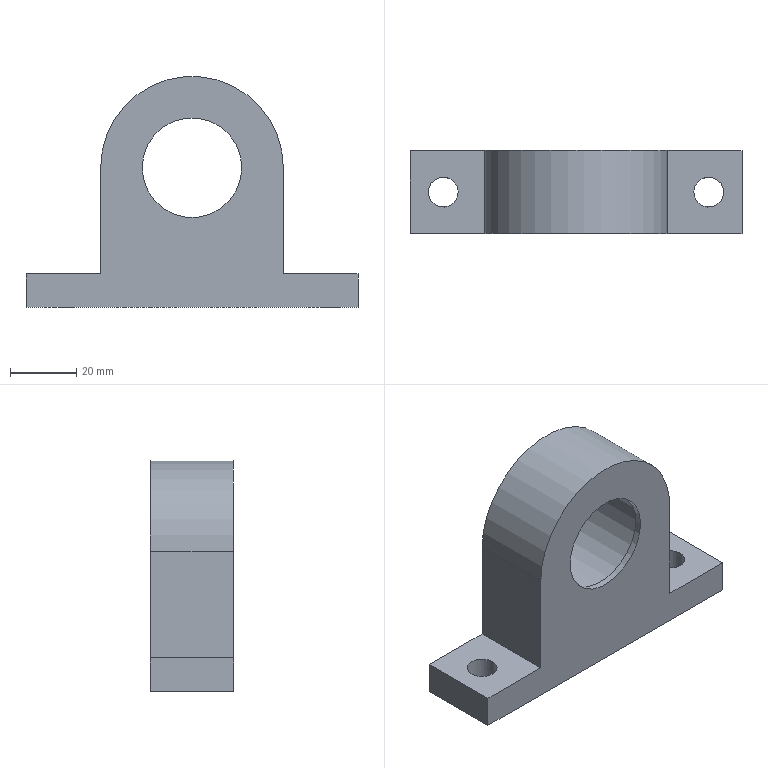Component | NX | BEARING_BLOCK_3 | 1 solid | 23 faces | volume 72548 mm3 | plane 14 | cylinder 9 | commonest cylinder face diameters 5 x4 9 x2 30 x1 55 x1 35 x1